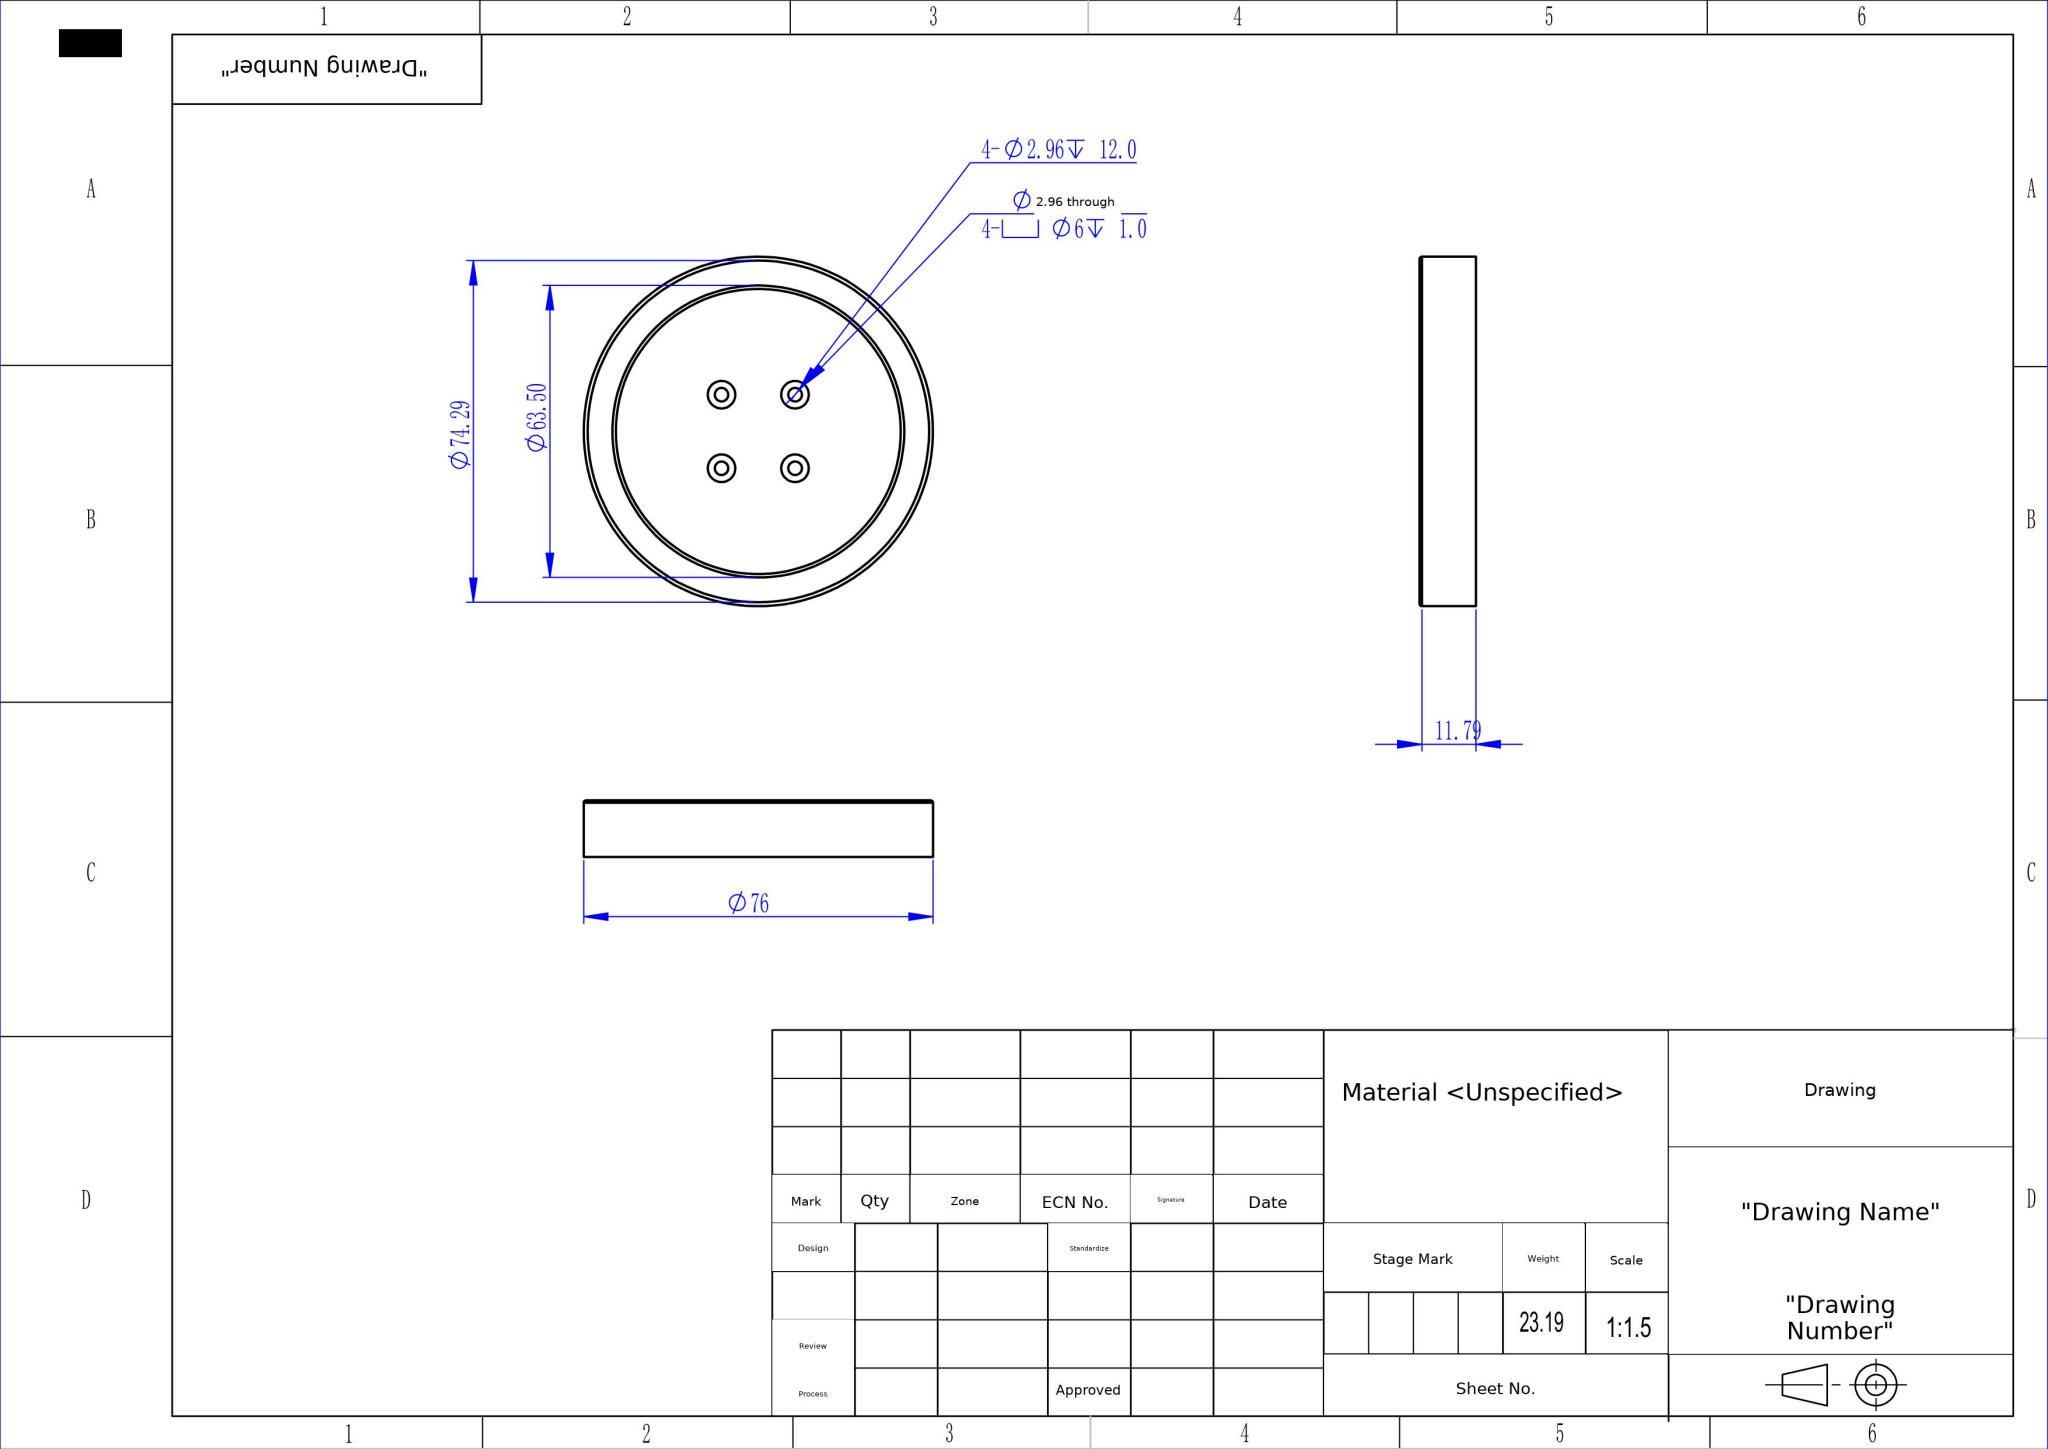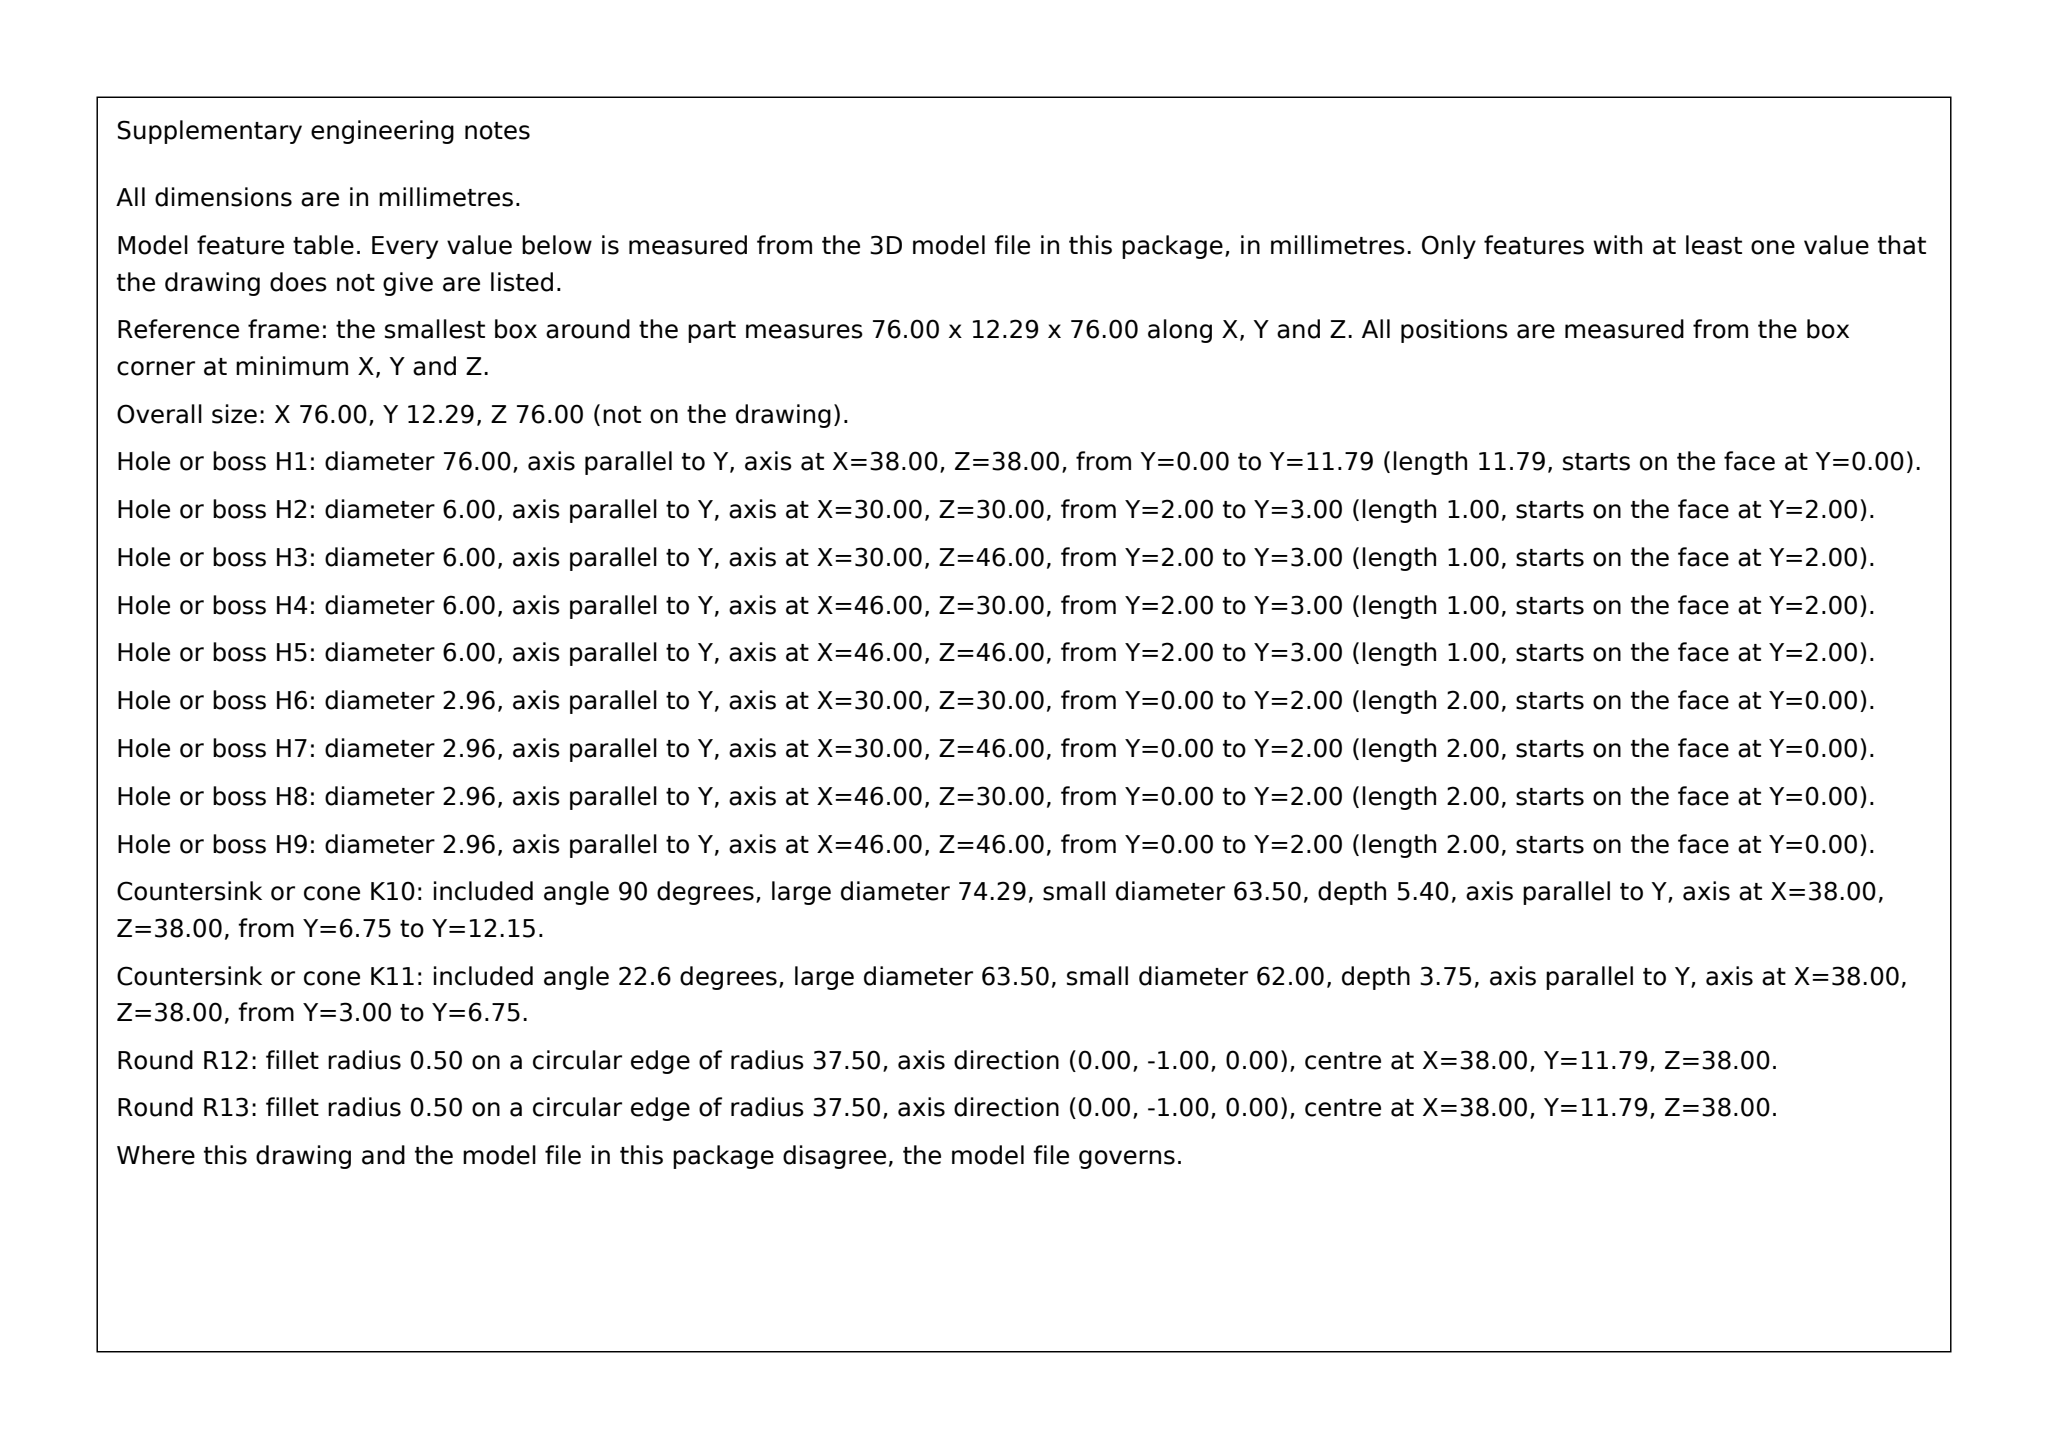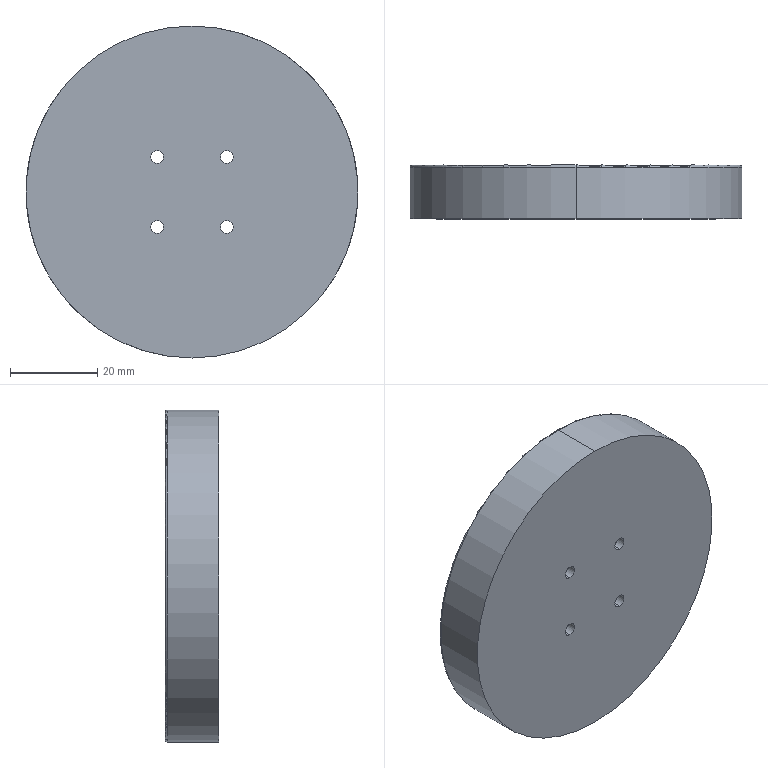Part | SolidWorks | mm | 1 solid | 30 faces | box 76 x 12.29 x 76 mm | volume 23190 mm3 | cylinder 18 | plane 6 | cone 4 | torus 2 | commonest cylinder face diameters 6 x8 2.956 x8 76 x2
STEP:
#1=CARTESIAN_POINT('',(0.,12.146,37.146));
#2=VERTEX_POINT('',#1);
#3=CARTESIAN_POINT('',(0.,12.146,-37.146));
#4=VERTEX_POINT('',#3);
#5=CARTESIAN_POINT('',(0.,12.146,0.));
#6=DIRECTION('',(0.,1.,0.));
#7=DIRECTION('',(0.,0.,1.));
#8=AXIS2_PLACEMENT_3D('',#5,#6,#7);
#9=CIRCLE('',#8,37.146);
#10=EDGE_CURVE('',#2,#4,#9,.T.);
#11=ORIENTED_EDGE('',*,*,#10,.F.);
#12=CARTESIAN_POINT('',(0.,11.793,38.));
#13=VERTEX_POINT('',#12);
#14=CARTESIAN_POINT('',(0.,11.793,37.5));
#15=DIRECTION('',(1.,0.,-0.));
#16=DIRECTION('',(-0.,0.,-1.));
#17=AXIS2_PLACEMENT_3D('',#14,#15,#16);
#18=CIRCLE('',#17,0.5);
#19=EDGE_CURVE('',#2,#13,#18,.T.);
#20=ORIENTED_EDGE('',*,*,#19,.T.);
#21=CARTESIAN_POINT('',(0.,11.793,-38.));
#22=VERTEX_POINT('',#21);
#23=CARTESIAN_POINT('',(0.,11.793,0.));
#24=DIRECTION('',(0.,-1.,0.));
#25=DIRECTION('',(0.,0.,-1.));
#26=AXIS2_PLACEMENT_3D('',#23,#24,#25);
#27=CIRCLE('',#26,38.);
#28=EDGE_CURVE('',#22,#13,#27,.T.);
#29=ORIENTED_EDGE('',*,*,#28,.F.);
#30=CARTESIAN_POINT('',(0.,11.793,-37.5));
#31=DIRECTION('',(-1.,0.,0.));
#32=DIRECTION('',(0.,0.,1.));
#33=AXIS2_PLACEMENT_3D('',#30,#31,#32);
#34=CIRCLE('',#33,0.5);
#35=EDGE_CURVE('',#4,#22,#34,.T.);
#36=ORIENTED_EDGE('',*,*,#35,.F.);
#37=EDGE_LOOP('',(#11,#20,#29,#36));
#38=FACE_OUTER_BOUND('',#37,.T.);
#39=CARTESIAN_POINT('',(0.,11.793,0.));
#40=DIRECTION('',(0.,-1.,0.));
#41=DIRECTION('',(0.,0.,-1.));
#42=AXIS2_PLACEMENT_3D('',#39,#40,#41);
#43=TOROIDAL_SURFACE('',#42,37.5,0.5);
#44=ADVANCED_FACE('',(#38),#43,.T.);
#45=CARTESIAN_POINT('',(0.,6.75,-31.75));
#46=VERTEX_POINT('',#45);
#47=CARTESIAN_POINT('',(0.,6.75,31.75));
#48=VERTEX_POINT('',#47);
#49=CARTESIAN_POINT('',(0.,6.75,0.));
#50=DIRECTION('',(0.,1.,0.));
#51=DIRECTION('',(0.,0.,1.));
#52=AXIS2_PLACEMENT_3D('',#49,#50,#51);
#53=CIRCLE('',#52,31.75);
#54=EDGE_CURVE('',#46,#48,#53,.T.);
#55=ORIENTED_EDGE('',*,*,#54,.F.);
#56=CARTESIAN_POINT('',(0.,6.75,-31.75));
#57=DIRECTION('',(0.,0.7071,-0.7071));
#58=VECTOR('',#57,1000.);
#59=LINE('',#56,#58);
#60=EDGE_CURVE('',#46,#4,#59,.T.);
#61=ORIENTED_EDGE('',*,*,#60,.T.);
#62=CARTESIAN_POINT('',(0.,12.146,0.));
#63=DIRECTION('',(0.,1.,0.));
#64=DIRECTION('',(0.,0.,1.));
#65=AXIS2_PLACEMENT_3D('',#62,#63,#64);
#66=CIRCLE('',#65,37.146);
#67=EDGE_CURVE('',#4,#2,#66,.T.);
#68=ORIENTED_EDGE('',*,*,#67,.T.);
#69=CARTESIAN_POINT('',(0.,6.75,31.75));
#70=DIRECTION('',(0.,0.7071,0.7071));
#71=VECTOR('',#70,1000.);
#72=LINE('',#69,#71);
#73=EDGE_CURVE('',#48,#2,#72,.T.);
#74=ORIENTED_EDGE('',*,*,#73,.F.);
#75=EDGE_LOOP('',(#55,#61,#68,#74));
#76=FACE_OUTER_BOUND('',#75,.T.);
#77=CARTESIAN_POINT('',(0.,6.75,0.));
#78=DIRECTION('',(0.,1.,0.));
#79=DIRECTION('',(0.,0.,1.));
#80=AXIS2_PLACEMENT_3D('',#77,#78,#79);
#81=CONICAL_SURFACE('',#80,31.75,0.7854);
#82=ADVANCED_FACE('',(#76),#81,.F.);
#83=CARTESIAN_POINT('',(0.,3.,-31.));
#84=VERTEX_POINT('',#83);
#85=CARTESIAN_POINT('',(0.,3.,31.));
#86=VERTEX_POINT('',#85);
#87=CARTESIAN_POINT('',(0.,3.,0.));
#88=DIRECTION('',(0.,1.,0.));
#89=DIRECTION('',(0.,0.,1.));
#90=AXIS2_PLACEMENT_3D('',#87,#88,#89);
#91=CIRCLE('',#90,31.);
#92=EDGE_CURVE('',#84,#86,#91,.T.);
#93=ORIENTED_EDGE('',*,*,#92,.F.);
#94=CARTESIAN_POINT('',(0.,13.,-33.));
#95=DIRECTION('',(0.,0.9806,-0.1961));
#96=VECTOR('',#95,1000.);
#97=LINE('',#94,#96);
#98=EDGE_CURVE('',#84,#46,#97,.T.);
#99=ORIENTED_EDGE('',*,*,#98,.T.);
#100=ORIENTED_EDGE('',*,*,#54,.T.);
#101=CARTESIAN_POINT('',(0.,13.,33.));
#102=DIRECTION('',(0.,0.9806,0.1961));
#103=VECTOR('',#102,1000.);
#104=LINE('',#101,#103);
#105=EDGE_CURVE('',#86,#48,#104,.T.);
#106=ORIENTED_EDGE('',*,*,#105,.F.);
#107=EDGE_LOOP('',(#93,#99,#100,#106));
#108=FACE_OUTER_BOUND('',#107,.T.);
#109=CARTESIAN_POINT('',(0.,13.,0.));
#110=DIRECTION('',(0.,1.,0.));
#111=DIRECTION('',(0.,0.,1.));
#112=AXIS2_PLACEMENT_3D('',#109,#110,#111);
#113=CONICAL_SURFACE('',#112,33.,0.1974);
#114=ADVANCED_FACE('',(#108),#113,.F.);
#115=CARTESIAN_POINT('',(-8.,2.,5.));
#116=VERTEX_POINT('',#115);
#117=CARTESIAN_POINT('',(-8.,2.,11.));
#118=VERTEX_POINT('',#117);
#119=CARTESIAN_POINT('',(-8.,2.,8.));
#120=DIRECTION('',(0.,1.,0.));
#121=DIRECTION('',(0.,0.,1.));
#122=AXIS2_PLACEMENT_3D('',#119,#120,#121);
#123=CIRCLE('',#122,3.);
#124=EDGE_CURVE('',#116,#118,#123,.T.);
#125=ORIENTED_EDGE('',*,*,#124,.F.);
#126=CARTESIAN_POINT('',(-8.,3.,5.));
#127=VERTEX_POINT('',#126);
#128=CARTESIAN_POINT('',(-8.,2.,5.));
#129=DIRECTION('',(0.,1.,0.));
#130=VECTOR('',#129,1000.);
#131=LINE('',#128,#130);
#132=EDGE_CURVE('',#116,#127,#131,.T.);
#133=ORIENTED_EDGE('',*,*,#132,.T.);
#134=CARTESIAN_POINT('',(-8.,3.,11.));
#135=VERTEX_POINT('',#134);
#136=CARTESIAN_POINT('',(-8.,3.,8.));
#137=DIRECTION('',(0.,1.,0.));
#138=DIRECTION('',(0.,0.,1.));
#139=AXIS2_PLACEMENT_3D('',#136,#137,#138);
#140=CIRCLE('',#139,3.);
#141=EDGE_CURVE('',#127,#135,#140,.T.);
#142=ORIENTED_EDGE('',*,*,#141,.T.);
#143=CARTESIAN_POINT('',(-8.,2.,11.));
#144=DIRECTION('',(0.,1.,0.));
#145=VECTOR('',#144,1000.);
#146=LINE('',#143,#145);
#147=EDGE_CURVE('',#118,#135,#146,.T.);
#148=ORIENTED_EDGE('',*,*,#147,.F.);
#149=EDGE_LOOP('',(#125,#133,#142,#148));
#150=FACE_OUTER_BOUND('',#149,.T.);
#151=CARTESIAN_POINT('',(-8.,2.,8.));
#152=DIRECTION('',(0.,1.,0.));
#153=DIRECTION('',(0.,0.,1.));
#154=AXIS2_PLACEMENT_3D('',#151,#152,#153);
#155=CYLINDRICAL_SURFACE('',#154,3.);
#156=ADVANCED_FACE('',(#150),#155,.F.);
#157=CARTESIAN_POINT('',(8.,2.,5.));
#158=VERTEX_POINT('',#157);
#159=CARTESIAN_POINT('',(8.,2.,11.));
#160=VERTEX_POINT('',#159);
#161=CARTESIAN_POINT('',(8.,2.,8.));
#162=DIRECTION('',(0.,1.,0.));
#163=DIRECTION('',(0.,0.,1.));
#164=AXIS2_PLACEMENT_3D('',#161,#162,#163);
#165=CIRCLE('',#164,3.);
#166=EDGE_CURVE('',#158,#160,#165,.T.);
#167=ORIENTED_EDGE('',*,*,#166,.F.);
#168=CARTESIAN_POINT('',(8.,3.,5.));
#169=VERTEX_POINT('',#168);
#170=CARTESIAN_POINT('',(8.,2.,5.));
#171=DIRECTION('',(0.,1.,0.));
#172=VECTOR('',#171,1000.);
#173=LINE('',#170,#172);
#174=EDGE_CURVE('',#158,#169,#173,.T.);
#175=ORIENTED_EDGE('',*,*,#174,.T.);
#176=CARTESIAN_POINT('',(8.,3.,11.));
#177=VERTEX_POINT('',#176);
#178=CARTESIAN_POINT('',(8.,3.,8.));
#179=DIRECTION('',(0.,1.,0.));
#180=DIRECTION('',(0.,0.,1.));
#181=AXIS2_PLACEMENT_3D('',#178,#179,#180);
#182=CIRCLE('',#181,3.);
#183=EDGE_CURVE('',#169,#177,#182,.T.);
#184=ORIENTED_EDGE('',*,*,#183,.T.);
#185=CARTESIAN_POINT('',(8.,2.,11.));
#186=DIRECTION('',(0.,1.,0.));
#187=VECTOR('',#186,1000.);
#188=LINE('',#185,#187);
#189=EDGE_CURVE('',#160,#177,#188,.T.);
#190=ORIENTED_EDGE('',*,*,#189,.F.);
#191=EDGE_LOOP('',(#167,#175,#184,#190));
#192=FACE_OUTER_BOUND('',#191,.T.);
#193=CARTESIAN_POINT('',(8.,2.,8.));
#194=DIRECTION('',(0.,1.,0.));
#195=DIRECTION('',(0.,0.,1.));
#196=AXIS2_PLACEMENT_3D('',#193,#194,#195);
#197=CYLINDRICAL_SURFACE('',#196,3.);
#198=ADVANCED_FACE('',(#192),#197,.F.);
#199=CARTESIAN_POINT('',(8.,2.,-11.));
#200=VERTEX_POINT('',#199);
#201=CARTESIAN_POINT('',(8.,2.,-5.));
#202=VERTEX_POINT('',#201);
#203=CARTESIAN_POINT('',(8.,2.,-8.));
#204=DIRECTION('',(0.,1.,0.));
#205=DIRECTION('',(0.,0.,1.));
#206=AXIS2_PLACEMENT_3D('',#203,#204,#205);
#207=CIRCLE('',#206,3.);
#208=EDGE_CURVE('',#200,#202,#207,.T.);
#209=ORIENTED_EDGE('',*,*,#208,.F.);
#210=CARTESIAN_POINT('',(8.,3.,-11.));
#211=VERTEX_POINT('',#210);
#212=CARTESIAN_POINT('',(8.,2.,-11.));
#213=DIRECTION('',(0.,1.,0.));
#214=VECTOR('',#213,1000.);
#215=LINE('',#212,#214);
#216=EDGE_CURVE('',#200,#211,#215,.T.);
#217=ORIENTED_EDGE('',*,*,#216,.T.);
#218=CARTESIAN_POINT('',(8.,3.,-5.));
#219=VERTEX_POINT('',#218);
#220=CARTESIAN_POINT('',(8.,3.,-8.));
#221=DIRECTION('',(0.,1.,0.));
#222=DIRECTION('',(0.,0.,1.));
#223=AXIS2_PLACEMENT_3D('',#220,#221,#222);
#224=CIRCLE('',#223,3.);
#225=EDGE_CURVE('',#211,#219,#224,.T.);
#226=ORIENTED_EDGE('',*,*,#225,.T.);
#227=CARTESIAN_POINT('',(8.,2.,-5.));
#228=DIRECTION('',(0.,1.,0.));
#229=VECTOR('',#228,1000.);
#230=LINE('',#227,#229);
#231=EDGE_CURVE('',#202,#219,#230,.T.);
#232=ORIENTED_EDGE('',*,*,#231,.F.);
#233=EDGE_LOOP('',(#209,#217,#226,#232));
#234=FACE_OUTER_BOUND('',#233,.T.);
#235=CARTESIAN_POINT('',(8.,2.,-8.));
#236=DIRECTION('',(0.,1.,0.));
#237=DIRECTION('',(0.,0.,1.));
#238=AXIS2_PLACEMENT_3D('',#235,#236,#237);
#239=CYLINDRICAL_SURFACE('',#238,3.);
#240=ADVANCED_FACE('',(#234),#239,.F.);
#241=CARTESIAN_POINT('',(-8.,2.,-11.));
#242=VERTEX_POINT('',#241);
#243=CARTESIAN_POINT('',(-8.,2.,-5.));
#244=VERTEX_POINT('',#243);
#245=CARTESIAN_POINT('',(-8.,2.,-8.));
#246=DIRECTION('',(0.,1.,0.));
#247=DIRECTION('',(0.,0.,1.));
#248=AXIS2_PLACEMENT_3D('',#245,#246,#247);
#249=CIRCLE('',#248,3.);
#250=EDGE_CURVE('',#242,#244,#249,.T.);
#251=ORIENTED_EDGE('',*,*,#250,.F.);
#252=CARTESIAN_POINT('',(-8.,3.,-11.));
#253=VERTEX_POINT('',#252);
#254=CARTESIAN_POINT('',(-8.,2.,-11.));
#255=DIRECTION('',(0.,1.,0.));
#256=VECTOR('',#255,1000.);
#257=LINE('',#254,#256);
#258=EDGE_CURVE('',#242,#253,#257,.T.);
#259=ORIENTED_EDGE('',*,*,#258,.T.);
#260=CARTESIAN_POINT('',(-8.,3.,-5.));
#261=VERTEX_POINT('',#260);
#262=CARTESIAN_POINT('',(-8.,3.,-8.));
#263=DIRECTION('',(0.,1.,0.));
#264=DIRECTION('',(0.,0.,1.));
#265=AXIS2_PLACEMENT_3D('',#262,#263,#264);
#266=CIRCLE('',#265,3.);
#267=EDGE_CURVE('',#253,#261,#266,.T.);
#268=ORIENTED_EDGE('',*,*,#267,.T.);
#269=CARTESIAN_POINT('',(-8.,2.,-5.));
#270=DIRECTION('',(0.,1.,0.));
#271=VECTOR('',#270,1000.);
#272=LINE('',#269,#271);
#273=EDGE_CURVE('',#244,#261,#272,.T.);
#274=ORIENTED_EDGE('',*,*,#273,.F.);
#275=EDGE_LOOP('',(#251,#259,#268,#274));
#276=FACE_OUTER_BOUND('',#275,.T.);
#277=CARTESIAN_POINT('',(-8.,2.,-8.));
#278=DIRECTION('',(0.,1.,0.));
#279=DIRECTION('',(0.,0.,1.));
#280=AXIS2_PLACEMENT_3D('',#277,#278,#279);
#281=CYLINDRICAL_SURFACE('',#280,3.);
#282=ADVANCED_FACE('',(#276),#281,.F.);
#283=ORIENTED_EDGE('',*,*,#28,.T.);
#284=CARTESIAN_POINT('',(0.,0.,38.));
#285=VERTEX_POINT('',#284);
#286=CARTESIAN_POINT('',(0.,3.,38.));
#287=DIRECTION('',(0.,-1.,0.));
#288=VECTOR('',#287,1000.);
#289=LINE('',#286,#288);
#290=EDGE_CURVE('',#13,#285,#289,.T.);
#291=ORIENTED_EDGE('',*,*,#290,.T.);
#292=CARTESIAN_POINT('',(0.,0.,-38.));
#293=VERTEX_POINT('',#292);
#294=CARTESIAN_POINT('',(0.,0.,0.));
#295=DIRECTION('',(0.,1.,0.));
#296=DIRECTION('',(0.,0.,1.));
#297=AXIS2_PLACEMENT_3D('',#294,#295,#296);
#298=CIRCLE('',#297,38.);
#299=EDGE_CURVE('',#285,#293,#298,.T.);
#300=ORIENTED_EDGE('',*,*,#299,.T.);
#301=CARTESIAN_POINT('',(0.,3.,-38.));
#302=DIRECTION('',(0.,-1.,0.));
#303=VECTOR('',#302,1000.);
#304=LINE('',#301,#303);
#305=EDGE_CURVE('',#22,#293,#304,.T.);
#306=ORIENTED_EDGE('',*,*,#305,.F.);
#307=EDGE_LOOP('',(#283,#291,#300,#306));
#308=FACE_OUTER_BOUND('',#307,.T.);
#309=CARTESIAN_POINT('',(0.,3.,0.));
#310=DIRECTION('',(0.,-1.,0.));
#311=DIRECTION('',(0.,0.,-1.));
#312=AXIS2_PLACEMENT_3D('',#309,#310,#311);
#313=CYLINDRICAL_SURFACE('',#312,38.);
#314=ADVANCED_FACE('',(#308),#313,.T.);
#315=CARTESIAN_POINT('',(-8.,0.,-9.478));
#316=VERTEX_POINT('',#315);
#317=CARTESIAN_POINT('',(-8.,0.,-6.522));
#318=VERTEX_POINT('',#317);
#319=CARTESIAN_POINT('',(-8.,0.,-8.));
#320=DIRECTION('',(0.,1.,0.));
#321=DIRECTION('',(0.,0.,1.));
#322=AXIS2_PLACEMENT_3D('',#319,#320,#321);
#323=CIRCLE('',#322,1.478);
#324=EDGE_CURVE('',#316,#318,#323,.T.);
#325=ORIENTED_EDGE('',*,*,#324,.F.);
#326=CARTESIAN_POINT('',(-8.,2.,-9.478));
#327=VERTEX_POINT('',#326);
#328=CARTESIAN_POINT('',(-8.,-9.,-9.478));
#329=DIRECTION('',(0.,1.,0.));
#330=VECTOR('',#329,1000.);
#331=LINE('',#328,#330);
#332=EDGE_CURVE('',#316,#327,#331,.T.);
#333=ORIENTED_EDGE('',*,*,#332,.T.);
#334=CARTESIAN_POINT('',(-8.,2.,-6.522));
#335=VERTEX_POINT('',#334);
#336=CARTESIAN_POINT('',(-8.,2.,-8.));
#337=DIRECTION('',(0.,-1.,0.));
#338=DIRECTION('',(0.,0.,1.));
#339=AXIS2_PLACEMENT_3D('',#336,#337,#338);
#340=CIRCLE('',#339,1.478);
#341=EDGE_CURVE('',#335,#327,#340,.T.);
#342=ORIENTED_EDGE('',*,*,#341,.F.);
#343=CARTESIAN_POINT('',(-8.,-9.,-6.522));
#344=DIRECTION('',(0.,1.,0.));
#345=VECTOR('',#344,1000.);
#346=LINE('',#343,#345);
#347=EDGE_CURVE('',#318,#335,#346,.T.);
#348=ORIENTED_EDGE('',*,*,#347,.F.);
#349=EDGE_LOOP('',(#325,#333,#342,#348));
#350=FACE_OUTER_BOUND('',#349,.T.);
#351=CARTESIAN_POINT('',(-8.,-9.,-8.));
#352=DIRECTION('',(0.,1.,0.));
#353=DIRECTION('',(0.,0.,1.));
#354=AXIS2_PLACEMENT_3D('',#351,#352,#353);
#355=CYLINDRICAL_SURFACE('',#354,1.478);
#356=ADVANCED_FACE('',(#350),#355,.F.);
#357=CARTESIAN_POINT('',(8.,0.,-9.478));
#358=VERTEX_POINT('',#357);
#359=CARTESIAN_POINT('',(8.,0.,-6.522));
#360=VERTEX_POINT('',#359);
#361=CARTESIAN_POINT('',(8.,0.,-8.));
#362=DIRECTION('',(0.,1.,0.));
#363=DIRECTION('',(0.,0.,1.));
#364=AXIS2_PLACEMENT_3D('',#361,#362,#363);
#365=CIRCLE('',#364,1.478);
#366=EDGE_CURVE('',#358,#360,#365,.T.);
#367=ORIENTED_EDGE('',*,*,#366,.F.);
#368=CARTESIAN_POINT('',(8.,2.,-9.478));
#369=VERTEX_POINT('',#368);
#370=CARTESIAN_POINT('',(8.,-9.,-9.478));
#371=DIRECTION('',(0.,1.,0.));
#372=VECTOR('',#371,1000.);
#373=LINE('',#370,#372);
#374=EDGE_CURVE('',#358,#369,#373,.T.);
#375=ORIENTED_EDGE('',*,*,#374,.T.);
#376=CARTESIAN_POINT('',(8.,2.,-6.522));
#377=VERTEX_POINT('',#376);
#378=CARTESIAN_POINT('',(8.,2.,-8.));
#379=DIRECTION('',(0.,-1.,0.));
#380=DIRECTION('',(0.,0.,1.));
#381=AXIS2_PLACEMENT_3D('',#378,#379,#380);
#382=CIRCLE('',#381,1.478);
#383=EDGE_CURVE('',#377,#369,#382,.T.);
#384=ORIENTED_EDGE('',*,*,#383,.F.);
#385=CARTESIAN_POINT('',(8.,-9.,-6.522));
#386=DIRECTION('',(0.,1.,0.));
#387=VECTOR('',#386,1000.);
#388=LINE('',#385,#387);
#389=EDGE_CURVE('',#360,#377,#388,.T.);
#390=ORIENTED_EDGE('',*,*,#389,.F.);
#391=EDGE_LOOP('',(#367,#375,#384,#390));
#392=FACE_OUTER_BOUND('',#391,.T.);
#393=CARTESIAN_POINT('',(8.,-9.,-8.));
#394=DIRECTION('',(0.,1.,0.));
#395=DIRECTION('',(0.,0.,1.));
#396=AXIS2_PLACEMENT_3D('',#393,#394,#395);
#397=CYLINDRICAL_SURFACE('',#396,1.478);
#398=ADVANCED_FACE('',(#392),#397,.F.);
#399=CARTESIAN_POINT('',(8.,0.,6.522));
#400=VERTEX_POINT('',#399);
#401=CARTESIAN_POINT('',(8.,0.,9.478));
#402=VERTEX_POINT('',#401);
#403=CARTESIAN_POINT('',(8.,0.,8.));
#404=DIRECTION('',(0.,1.,0.));
#405=DIRECTION('',(0.,0.,1.));
#406=AXIS2_PLACEMENT_3D('',#403,#404,#405);
#407=CIRCLE('',#406,1.478);
#408=EDGE_CURVE('',#400,#402,#407,.T.);
#409=ORIENTED_EDGE('',*,*,#408,.F.);
#410=CARTESIAN_POINT('',(8.,2.,6.522));
#411=VERTEX_POINT('',#410);
#412=CARTESIAN_POINT('',(8.,-9.,6.522));
#413=DIRECTION('',(0.,1.,0.));
#414=VECTOR('',#413,1000.);
#415=LINE('',#412,#414);
#416=EDGE_CURVE('',#400,#411,#415,.T.);
#417=ORIENTED_EDGE('',*,*,#416,.T.);
#418=CARTESIAN_POINT('',(8.,2.,9.478));
#419=VERTEX_POINT('',#418);
#420=CARTESIAN_POINT('',(8.,2.,8.));
#421=DIRECTION('',(0.,-1.,0.));
#422=DIRECTION('',(0.,0.,1.));
#423=AXIS2_PLACEMENT_3D('',#420,#421,#422);
#424=CIRCLE('',#423,1.478);
#425=EDGE_CURVE('',#419,#411,#424,.T.);
#426=ORIENTED_EDGE('',*,*,#425,.F.);
#427=CARTESIAN_POINT('',(8.,-9.,9.478));
#428=DIRECTION('',(0.,1.,0.));
#429=VECTOR('',#428,1000.);
#430=LINE('',#427,#429);
#431=EDGE_CURVE('',#402,#419,#430,.T.);
#432=ORIENTED_EDGE('',*,*,#431,.F.);
#433=EDGE_LOOP('',(#409,#417,#426,#432));
#434=FACE_OUTER_BOUND('',#433,.T.);
#435=CARTESIAN_POINT('',(8.,-9.,8.));
#436=DIRECTION('',(0.,1.,0.));
#437=DIRECTION('',(0.,0.,1.));
#438=AXIS2_PLACEMENT_3D('',#435,#436,#437);
#439=CYLINDRICAL_SURFACE('',#438,1.478);
#440=ADVANCED_FACE('',(#434),#439,.F.);
#441=CARTESIAN_POINT('',(-8.,0.,6.522));
#442=VERTEX_POINT('',#441);
#443=CARTESIAN_POINT('',(-8.,0.,9.478));
#444=VERTEX_POINT('',#443);
#445=CARTESIAN_POINT('',(-8.,0.,8.));
#446=DIRECTION('',(0.,1.,0.));
#447=DIRECTION('',(0.,0.,1.));
#448=AXIS2_PLACEMENT_3D('',#445,#446,#447);
#449=CIRCLE('',#448,1.478);
#450=EDGE_CURVE('',#442,#444,#449,.T.);
#451=ORIENTED_EDGE('',*,*,#450,.F.);
#452=CARTESIAN_POINT('',(-8.,2.,6.522));
#453=VERTEX_POINT('',#452);
#454=CARTESIAN_POINT('',(-8.,-9.,6.522));
#455=DIRECTION('',(0.,1.,0.));
#456=VECTOR('',#455,1000.);
#457=LINE('',#454,#456);
#458=EDGE_CURVE('',#442,#453,#457,.T.);
#459=ORIENTED_EDGE('',*,*,#458,.T.);
#460=CARTESIAN_POINT('',(-8.,2.,9.478));
#461=VERTEX_POINT('',#460);
#462=CARTESIAN_POINT('',(-8.,2.,8.));
#463=DIRECTION('',(0.,-1.,0.));
#464=DIRECTION('',(0.,0.,1.));
#465=AXIS2_PLACEMENT_3D('',#462,#463,#464);
#466=CIRCLE('',#465,1.478);
#467=EDGE_CURVE('',#461,#453,#466,.T.);
#468=ORIENTED_EDGE('',*,*,#467,.F.);
#469=CARTESIAN_POINT('',(-8.,-9.,9.478));
#470=DIRECTION('',(0.,1.,0.));
#471=VECTOR('',#470,1000.);
#472=LINE('',#469,#471);
#473=EDGE_CURVE('',#444,#461,#472,.T.);
#474=ORIENTED_EDGE('',*,*,#473,.F.);
#475=EDGE_LOOP('',(#451,#459,#468,#474));
#476=FACE_OUTER_BOUND('',#475,.T.);
#477=CARTESIAN_POINT('',(-8.,-9.,8.));
#478=DIRECTION('',(0.,1.,0.));
#479=DIRECTION('',(0.,0.,1.));
#480=AXIS2_PLACEMENT_3D('',#477,#478,#479);
#481=CYLINDRICAL_SURFACE('',#480,1.478);
#482=ADVANCED_FACE('',(#476),#481,.F.);
#483=ORIENTED_EDGE('',*,*,#458,.F.);
#484=CARTESIAN_POINT('',(-8.,0.,8.));
#485=DIRECTION('',(0.,1.,0.));
#486=DIRECTION('',(0.,0.,1.));
#487=AXIS2_PLACEMENT_3D('',#484,#485,#486);
#488=CIRCLE('',#487,1.478);
#489=EDGE_CURVE('',#444,#442,#488,.T.);
#490=ORIENTED_EDGE('',*,*,#489,.F.);
#491=ORIENTED_EDGE('',*,*,#473,.T.);
#492=CARTESIAN_POINT('',(-8.,2.,8.));
#493=DIRECTION('',(0.,-1.,0.));
#494=DIRECTION('',(0.,0.,1.));
#495=AXIS2_PLACEMENT_3D('',#492,#493,#494);
#496=CIRCLE('',#495,1.478);
#497=EDGE_CURVE('',#453,#461,#496,.T.);
#498=ORIENTED_EDGE('',*,*,#497,.F.);
#499=EDGE_LOOP('',(#483,#490,#491,#498));
#500=FACE_OUTER_BOUND('',#499,.T.);
#501=CARTESIAN_POINT('',(-8.,-9.,8.));
#502=DIRECTION('',(0.,1.,0.));
#503=DIRECTION('',(0.,0.,1.));
#504=AXIS2_PLACEMENT_3D('',#501,#502,#503);
#505=CYLINDRICAL_SURFACE('',#504,1.478);
#506=ADVANCED_FACE('',(#500),#505,.F.);
#507=ORIENTED_EDGE('',*,*,#416,.F.);
#508=CARTESIAN_POINT('',(8.,0.,8.));
#509=DIRECTION('',(0.,1.,0.));
#510=DIRECTION('',(0.,0.,1.));
#511=AXIS2_PLACEMENT_3D('',#508,#509,#510);
#512=CIRCLE('',#511,1.478);
#513=EDGE_CURVE('',#402,#400,#512,.T.);
#514=ORIENTED_EDGE('',*,*,#513,.F.);
#515=ORIENTED_EDGE('',*,*,#431,.T.);
#516=CARTESIAN_POINT('',(8.,2.,8.));
#517=DIRECTION('',(0.,-1.,0.));
#518=DIRECTION('',(0.,0.,1.));
#519=AXIS2_PLACEMENT_3D('',#516,#517,#518);
#520=CIRCLE('',#519,1.478);
#521=EDGE_CURVE('',#411,#419,#520,.T.);
#522=ORIENTED_EDGE('',*,*,#521,.F.);
#523=EDGE_LOOP('',(#507,#514,#515,#522));
#524=FACE_OUTER_BOUND('',#523,.T.);
#525=CARTESIAN_POINT('',(8.,-9.,8.));
#526=DIRECTION('',(0.,1.,0.));
#527=DIRECTION('',(0.,0.,1.));
#528=AXIS2_PLACEMENT_3D('',#525,#526,#527);
#529=CYLINDRICAL_SURFACE('',#528,1.478);
#530=ADVANCED_FACE('',(#524),#529,.F.);
#531=ORIENTED_EDGE('',*,*,#374,.F.);
#532=CARTESIAN_POINT('',(8.,0.,-8.));
#533=DIRECTION('',(0.,1.,0.));
#534=DIRECTION('',(0.,0.,1.));
#535=AXIS2_PLACEMENT_3D('',#532,#533,#534);
#536=CIRCLE('',#535,1.478);
#537=EDGE_CURVE('',#360,#358,#536,.T.);
#538=ORIENTED_EDGE('',*,*,#537,.F.);
#539=ORIENTED_EDGE('',*,*,#389,.T.);
#540=CARTESIAN_POINT('',(8.,2.,-8.));
#541=DIRECTION('',(0.,-1.,0.));
#542=DIRECTION('',(0.,0.,1.));
#543=AXIS2_PLACEMENT_3D('',#540,#541,#542);
#544=CIRCLE('',#543,1.478);
#545=EDGE_CURVE('',#369,#377,#544,.T.);
#546=ORIENTED_EDGE('',*,*,#545,.F.);
#547=EDGE_LOOP('',(#531,#538,#539,#546));
#548=FACE_OUTER_BOUND('',#547,.T.);
#549=CARTESIAN_POINT('',(8.,-9.,-8.));
#550=DIRECTION('',(0.,1.,0.));
#551=DIRECTION('',(0.,0.,1.));
#552=AXIS2_PLACEMENT_3D('',#549,#550,#551);
#553=CYLINDRICAL_SURFACE('',#552,1.478);
#554=ADVANCED_FACE('',(#548),#553,.F.);
#555=ORIENTED_EDGE('',*,*,#332,.F.);
#556=CARTESIAN_POINT('',(-8.,0.,-8.));
#557=DIRECTION('',(0.,1.,0.));
#558=DIRECTION('',(0.,0.,1.));
#559=AXIS2_PLACEMENT_3D('',#556,#557,#558);
#560=CIRCLE('',#559,1.478);
#561=EDGE_CURVE('',#318,#316,#560,.T.);
#562=ORIENTED_EDGE('',*,*,#561,.F.);
#563=ORIENTED_EDGE('',*,*,#347,.T.);
#564=CARTESIAN_POINT('',(-8.,2.,-8.));
#565=DIRECTION('',(0.,-1.,0.));
#566=DIRECTION('',(0.,0.,1.));
#567=AXIS2_PLACEMENT_3D('',#564,#565,#566);
#568=CIRCLE('',#567,1.478);
#569=EDGE_CURVE('',#327,#335,#568,.T.);
#570=ORIENTED_EDGE('',*,*,#569,.F.);
#571=EDGE_LOOP('',(#555,#562,#563,#570));
#572=FACE_OUTER_BOUND('',#571,.T.);
#573=CARTESIAN_POINT('',(-8.,-9.,-8.));
#574=DIRECTION('',(0.,1.,0.));
#575=DIRECTION('',(0.,0.,1.));
#576=AXIS2_PLACEMENT_3D('',#573,#574,#575);
#577=CYLINDRICAL_SURFACE('',#576,1.478);
#578=ADVANCED_FACE('',(#572),#577,.F.);
#579=ORIENTED_EDGE('',*,*,#290,.F.);
#580=CARTESIAN_POINT('',(0.,11.793,0.));
#581=DIRECTION('',(0.,-1.,0.));
#582=DIRECTION('',(0.,0.,-1.));
#583=AXIS2_PLACEMENT_3D('',#580,#581,#582);
#584=CIRCLE('',#583,38.);
#585=EDGE_CURVE('',#13,#22,#584,.T.);
#586=ORIENTED_EDGE('',*,*,#585,.T.);
#587=ORIENTED_EDGE('',*,*,#305,.T.);
#588=CARTESIAN_POINT('',(0.,0.,0.));
#589=DIRECTION('',(0.,1.,0.));
#590=DIRECTION('',(0.,0.,1.));
#591=AXIS2_PLACEMENT_3D('',#588,#589,#590);
#592=CIRCLE('',#591,38.);
#593=EDGE_CURVE('',#293,#285,#592,.T.);
#594=ORIENTED_EDGE('',*,*,#593,.T.);
#595=EDGE_LOOP('',(#579,#586,#587,#594));
#596=FACE_OUTER_BOUND('',#595,.T.);
#597=CARTESIAN_POINT('',(0.,3.,0.));
#598=DIRECTION('',(0.,-1.,0.));
#599=DIRECTION('',(0.,0.,-1.));
#600=AXIS2_PLACEMENT_3D('',#597,#598,#599);
#601=CYLINDRICAL_SURFACE('',#600,38.);
#602=ADVANCED_FACE('',(#596),#601,.T.);
#603=ORIENTED_EDGE('',*,*,#561,.T.);
#604=ORIENTED_EDGE('',*,*,#324,.T.);
#605=EDGE_LOOP('',(#603,#604));
#606=FACE_BOUND('',#605,.T.);
#607=ORIENTED_EDGE('',*,*,#537,.T.);
#608=ORIENTED_EDGE('',*,*,#366,.T.);
#609=EDGE_LOOP('',(#607,#608));
#610=FACE_BOUND('',#609,.T.);
#611=ORIENTED_EDGE('',*,*,#513,.T.);
#612=ORIENTED_EDGE('',*,*,#408,.T.);
#613=EDGE_LOOP('',(#611,#612));
#614=FACE_BOUND('',#613,.T.);
#615=ORIENTED_EDGE('',*,*,#489,.T.);
#616=ORIENTED_EDGE('',*,*,#450,.T.);
#617=EDGE_LOOP('',(#615,#616));
#618=FACE_BOUND('',#617,.T.);
#619=ORIENTED_EDGE('',*,*,#593,.F.);
#620=ORIENTED_EDGE('',*,*,#299,.F.);
#621=EDGE_LOOP('',(#619,#620));
#622=FACE_OUTER_BOUND('',#621,.T.);
#623=CARTESIAN_POINT('',(0.,0.,0.));
#624=DIRECTION('',(0.,1.,0.));
#625=DIRECTION('',(0.,0.,1.));
#626=AXIS2_PLACEMENT_3D('',#623,#624,#625);
#627=PLANE('',#626);
#628=ADVANCED_FACE('',(#606,#610,#614,#618,#622),#627,.F.);
#629=CARTESIAN_POINT('',(0.,3.,0.));
#630=DIRECTION('',(0.,1.,0.));
#631=DIRECTION('',(0.,0.,1.));
#632=AXIS2_PLACEMENT_3D('',#629,#630,#631);
#633=CIRCLE('',#632,31.);
#634=EDGE_CURVE('',#86,#84,#633,.T.);
#635=ORIENTED_EDGE('',*,*,#634,.T.);
#636=ORIENTED_EDGE('',*,*,#92,.T.);
#637=EDGE_LOOP('',(#635,#636));
#638=FACE_OUTER_BOUND('',#637,.T.);
#639=CARTESIAN_POINT('',(-8.,3.,8.));
#640=DIRECTION('',(0.,1.,0.));
#641=DIRECTION('',(0.,0.,1.));
#642=AXIS2_PLACEMENT_3D('',#639,#640,#641);
#643=CIRCLE('',#642,3.);
#644=EDGE_CURVE('',#135,#127,#643,.T.);
#645=ORIENTED_EDGE('',*,*,#644,.F.);
#646=ORIENTED_EDGE('',*,*,#141,.F.);
#647=EDGE_LOOP('',(#645,#646));
#648=FACE_BOUND('',#647,.T.);
#649=CARTESIAN_POINT('',(8.,3.,8.));
#650=DIRECTION('',(0.,1.,0.));
#651=DIRECTION('',(0.,0.,1.));
#652=AXIS2_PLACEMENT_3D('',#649,#650,#651);
#653=CIRCLE('',#652,3.);
#654=EDGE_CURVE('',#177,#169,#653,.T.);
#655=ORIENTED_EDGE('',*,*,#654,.F.);
#656=ORIENTED_EDGE('',*,*,#183,.F.);
#657=EDGE_LOOP('',(#655,#656));
#658=FACE_BOUND('',#657,.T.);
#659=CARTESIAN_POINT('',(8.,3.,-8.));
#660=DIRECTION('',(0.,1.,0.));
#661=DIRECTION('',(0.,0.,1.));
#662=AXIS2_PLACEMENT_3D('',#659,#660,#661);
#663=CIRCLE('',#662,3.);
#664=EDGE_CURVE('',#219,#211,#663,.T.);
#665=ORIENTED_EDGE('',*,*,#664,.F.);
#666=ORIENTED_EDGE('',*,*,#225,.F.);
#667=EDGE_LOOP('',(#665,#666));
#668=FACE_BOUND('',#667,.T.);
#669=CARTESIAN_POINT('',(-8.,3.,-8.));
#670=DIRECTION('',(0.,1.,0.));
#671=DIRECTION('',(0.,0.,1.));
#672=AXIS2_PLACEMENT_3D('',#669,#670,#671);
#673=CIRCLE('',#672,3.);
#674=EDGE_CURVE('',#261,#253,#673,.T.);
#675=ORIENTED_EDGE('',*,*,#674,.F.);
#676=ORIENTED_EDGE('',*,*,#267,.F.);
#677=EDGE_LOOP('',(#675,#676));
#678=FACE_BOUND('',#677,.T.);
#679=CARTESIAN_POINT('',(0.,3.,0.));
#680=DIRECTION('',(0.,1.,0.));
#681=DIRECTION('',(0.,0.,1.));
#682=AXIS2_PLACEMENT_3D('',#679,#680,#681);
#683=PLANE('',#682);
#684=ADVANCED_FACE('',(#638,#648,#658,#668,#678),#683,.T.);
#685=CARTESIAN_POINT('',(-8.,2.,-8.));
#686=DIRECTION('',(0.,1.,0.));
#687=DIRECTION('',(0.,0.,1.));
#688=AXIS2_PLACEMENT_3D('',#685,#686,#687);
#689=CIRCLE('',#688,3.);
#690=EDGE_CURVE('',#244,#242,#689,.T.);
#691=ORIENTED_EDGE('',*,*,#690,.T.);
#692=ORIENTED_EDGE('',*,*,#250,.T.);
#693=EDGE_LOOP('',(#691,#692));
#694=FACE_OUTER_BOUND('',#693,.T.);
#695=ORIENTED_EDGE('',*,*,#341,.T.);
#696=ORIENTED_EDGE('',*,*,#569,.T.);
#697=EDGE_LOOP('',(#695,#696));
#698=FACE_BOUND('',#697,.T.);
#699=CARTESIAN_POINT('',(-8.,2.,-8.));
#700=DIRECTION('',(0.,1.,0.));
#701=DIRECTION('',(0.,0.,1.));
#702=AXIS2_PLACEMENT_3D('',#699,#700,#701);
#703=PLANE('',#702);
#704=ADVANCED_FACE('',(#694,#698),#703,.T.);
#705=ORIENTED_EDGE('',*,*,#258,.F.);
#706=ORIENTED_EDGE('',*,*,#690,.F.);
#707=ORIENTED_EDGE('',*,*,#273,.T.);
#708=ORIENTED_EDGE('',*,*,#674,.T.);
#709=EDGE_LOOP('',(#705,#706,#707,#708));
#710=FACE_OUTER_BOUND('',#709,.T.);
#711=CARTESIAN_POINT('',(-8.,2.,-8.));
#712=DIRECTION('',(0.,1.,0.));
#713=DIRECTION('',(0.,0.,1.));
#714=AXIS2_PLACEMENT_3D('',#711,#712,#713);
#715=CYLINDRICAL_SURFACE('',#714,3.);
#716=ADVANCED_FACE('',(#710),#715,.F.);
#717=CARTESIAN_POINT('',(8.,2.,-8.));
#718=DIRECTION('',(0.,1.,0.));
#719=DIRECTION('',(0.,0.,1.));
#720=AXIS2_PLACEMENT_3D('',#717,#718,#719);
#721=CIRCLE('',#720,3.);
#722=EDGE_CURVE('',#202,#200,#721,.T.);
#723=ORIENTED_EDGE('',*,*,#722,.T.);
#724=ORIENTED_EDGE('',*,*,#208,.T.);
#725=EDGE_LOOP('',(#723,#724));
#726=FACE_OUTER_BOUND('',#725,.T.);
#727=ORIENTED_EDGE('',*,*,#383,.T.);
#728=ORIENTED_EDGE('',*,*,#545,.T.);
#729=EDGE_LOOP('',(#727,#728));
#730=FACE_BOUND('',#729,.T.);
#731=CARTESIAN_POINT('',(8.,2.,-8.));
#732=DIRECTION('',(0.,1.,0.));
#733=DIRECTION('',(0.,0.,1.));
#734=AXIS2_PLACEMENT_3D('',#731,#732,#733);
#735=PLANE('',#734);
#736=ADVANCED_FACE('',(#726,#730),#735,.T.);
#737=ORIENTED_EDGE('',*,*,#216,.F.);
#738=ORIENTED_EDGE('',*,*,#722,.F.);
#739=ORIENTED_EDGE('',*,*,#231,.T.);
#740=ORIENTED_EDGE('',*,*,#664,.T.);
#741=EDGE_LOOP('',(#737,#738,#739,#740));
#742=FACE_OUTER_BOUND('',#741,.T.);
#743=CARTESIAN_POINT('',(8.,2.,-8.));
#744=DIRECTION('',(0.,1.,0.));
#745=DIRECTION('',(0.,0.,1.));
#746=AXIS2_PLACEMENT_3D('',#743,#744,#745);
#747=CYLINDRICAL_SURFACE('',#746,3.);
#748=ADVANCED_FACE('',(#742),#747,.F.);
#749=CARTESIAN_POINT('',(8.,2.,8.));
#750=DIRECTION('',(0.,1.,0.));
#751=DIRECTION('',(0.,0.,1.));
#752=AXIS2_PLACEMENT_3D('',#749,#750,#751);
#753=CIRCLE('',#752,3.);
#754=EDGE_CURVE('',#160,#158,#753,.T.);
#755=ORIENTED_EDGE('',*,*,#754,.T.);
#756=ORIENTED_EDGE('',*,*,#166,.T.);
#757=EDGE_LOOP('',(#755,#756));
#758=FACE_OUTER_BOUND('',#757,.T.);
#759=ORIENTED_EDGE('',*,*,#425,.T.);
#760=ORIENTED_EDGE('',*,*,#521,.T.);
#761=EDGE_LOOP('',(#759,#760));
#762=FACE_BOUND('',#761,.T.);
#763=CARTESIAN_POINT('',(8.,2.,8.));
#764=DIRECTION('',(0.,1.,0.));
#765=DIRECTION('',(0.,0.,1.));
#766=AXIS2_PLACEMENT_3D('',#763,#764,#765);
#767=PLANE('',#766);
#768=ADVANCED_FACE('',(#758,#762),#767,.T.);
#769=ORIENTED_EDGE('',*,*,#174,.F.);
#770=ORIENTED_EDGE('',*,*,#754,.F.);
#771=ORIENTED_EDGE('',*,*,#189,.T.);
#772=ORIENTED_EDGE('',*,*,#654,.T.);
#773=EDGE_LOOP('',(#769,#770,#771,#772));
#774=FACE_OUTER_BOUND('',#773,.T.);
#775=CARTESIAN_POINT('',(8.,2.,8.));
#776=DIRECTION('',(0.,1.,0.));
#777=DIRECTION('',(0.,0.,1.));
#778=AXIS2_PLACEMENT_3D('',#775,#776,#777);
#779=CYLINDRICAL_SURFACE('',#778,3.);
#780=ADVANCED_FACE('',(#774),#779,.F.);
#781=CARTESIAN_POINT('',(-8.,2.,8.));
#782=DIRECTION('',(0.,1.,0.));
#783=DIRECTION('',(0.,0.,1.));
#784=AXIS2_PLACEMENT_3D('',#781,#782,#783);
#785=CIRCLE('',#784,3.);
#786=EDGE_CURVE('',#118,#116,#785,.T.);
#787=ORIENTED_EDGE('',*,*,#786,.T.);
#788=ORIENTED_EDGE('',*,*,#124,.T.);
#789=EDGE_LOOP('',(#787,#788));
#790=FACE_OUTER_BOUND('',#789,.T.);
#791=ORIENTED_EDGE('',*,*,#467,.T.);
#792=ORIENTED_EDGE('',*,*,#497,.T.);
#793=EDGE_LOOP('',(#791,#792));
#794=FACE_BOUND('',#793,.T.);
#795=CARTESIAN_POINT('',(-8.,2.,8.));
#796=DIRECTION('',(0.,1.,0.));
#797=DIRECTION('',(0.,0.,1.));
#798=AXIS2_PLACEMENT_3D('',#795,#796,#797);
#799=PLANE('',#798);
#800=ADVANCED_FACE('',(#790,#794),#799,.T.);
#801=ORIENTED_EDGE('',*,*,#132,.F.);
#802=ORIENTED_EDGE('',*,*,#786,.F.);
#803=ORIENTED_EDGE('',*,*,#147,.T.);
#804=ORIENTED_EDGE('',*,*,#644,.T.);
#805=EDGE_LOOP('',(#801,#802,#803,#804));
#806=FACE_OUTER_BOUND('',#805,.T.);
#807=CARTESIAN_POINT('',(-8.,2.,8.));
#808=DIRECTION('',(0.,1.,0.));
#809=DIRECTION('',(0.,0.,1.));
#810=AXIS2_PLACEMENT_3D('',#807,#808,#809);
#811=CYLINDRICAL_SURFACE('',#810,3.);
#812=ADVANCED_FACE('',(#806),#811,.F.);
#813=ORIENTED_EDGE('',*,*,#98,.F.);
#814=ORIENTED_EDGE('',*,*,#634,.F.);
#815=ORIENTED_EDGE('',*,*,#105,.T.);
#816=CARTESIAN_POINT('',(0.,6.75,0.));
#817=DIRECTION('',(0.,1.,0.));
#818=DIRECTION('',(0.,0.,1.));
#819=AXIS2_PLACEMENT_3D('',#816,#817,#818);
#820=CIRCLE('',#819,31.75);
#821=EDGE_CURVE('',#48,#46,#820,.T.);
#822=ORIENTED_EDGE('',*,*,#821,.T.);
#823=EDGE_LOOP('',(#813,#814,#815,#822));
#824=FACE_OUTER_BOUND('',#823,.T.);
#825=CARTESIAN_POINT('',(0.,13.,0.));
#826=DIRECTION('',(0.,1.,0.));
#827=DIRECTION('',(0.,0.,1.));
#828=AXIS2_PLACEMENT_3D('',#825,#826,#827);
#829=CONICAL_SURFACE('',#828,33.,0.1974);
#830=ADVANCED_FACE('',(#824),#829,.F.);
#831=ORIENTED_EDGE('',*,*,#60,.F.);
#832=ORIENTED_EDGE('',*,*,#821,.F.);
#833=ORIENTED_EDGE('',*,*,#73,.T.);
#834=ORIENTED_EDGE('',*,*,#10,.T.);
#835=EDGE_LOOP('',(#831,#832,#833,#834));
#836=FACE_OUTER_BOUND('',#835,.T.);
#837=CARTESIAN_POINT('',(0.,6.75,0.));
#838=DIRECTION('',(0.,1.,0.));
#839=DIRECTION('',(0.,0.,1.));
#840=AXIS2_PLACEMENT_3D('',#837,#838,#839);
#841=CONICAL_SURFACE('',#840,31.75,0.7854);
#842=ADVANCED_FACE('',(#836),#841,.F.);
#843=ORIENTED_EDGE('',*,*,#19,.F.);
#844=ORIENTED_EDGE('',*,*,#67,.F.);
#845=ORIENTED_EDGE('',*,*,#35,.T.);
#846=ORIENTED_EDGE('',*,*,#585,.F.);
#847=EDGE_LOOP('',(#843,#844,#845,#846));
#848=FACE_OUTER_BOUND('',#847,.T.);
#849=CARTESIAN_POINT('',(0.,11.793,0.));
#850=DIRECTION('',(0.,-1.,0.));
#851=DIRECTION('',(0.,0.,-1.));
#852=AXIS2_PLACEMENT_3D('',#849,#850,#851);
#853=TOROIDAL_SURFACE('',#852,37.5,0.5);
#854=ADVANCED_FACE('',(#848),#853,.T.);
#855=CLOSED_SHELL('',(#44,#82,#114,#156,#198,#240,#282,#314,#356,#398,#440,#482,#506,#530,#554,#578,#602,#628,#684,#704,#716,#736,#748,#768,#780,#800,#812,#830,#842,#854));
#856=MANIFOLD_SOLID_BREP('',#855);
#857=CARTESIAN_POINT('',(0.,0.,0.));
#858=DIRECTION('',(0.,0.,1.));
#859=DIRECTION('',(1.,0.,0.));
#860=AXIS2_PLACEMENT_3D('',#857,#858,#859);
#861=(LENGTH_UNIT()NAMED_UNIT(*)SI_UNIT(.MILLI.,.METRE.));
#862=UNCERTAINTY_MEASURE_WITH_UNIT(LENGTH_MEASURE(0.00001),#861,'','');
#863=(NAMED_UNIT(*)PLANE_ANGLE_UNIT()SI_UNIT($,.RADIAN.));
#864=(NAMED_UNIT(*)SI_UNIT($,.STERADIAN.)SOLID_ANGLE_UNIT());
#865=(GEOMETRIC_REPRESENTATION_CONTEXT(3)GLOBAL_UNCERTAINTY_ASSIGNED_CONTEXT((#862))GLOBAL_UNIT_ASSIGNED_CONTEXT((#861,#863,#864))REPRESENTATION_CONTEXT('',''));
#866=ADVANCED_BREP_SHAPE_REPRESENTATION('',(#856,#860),#865);